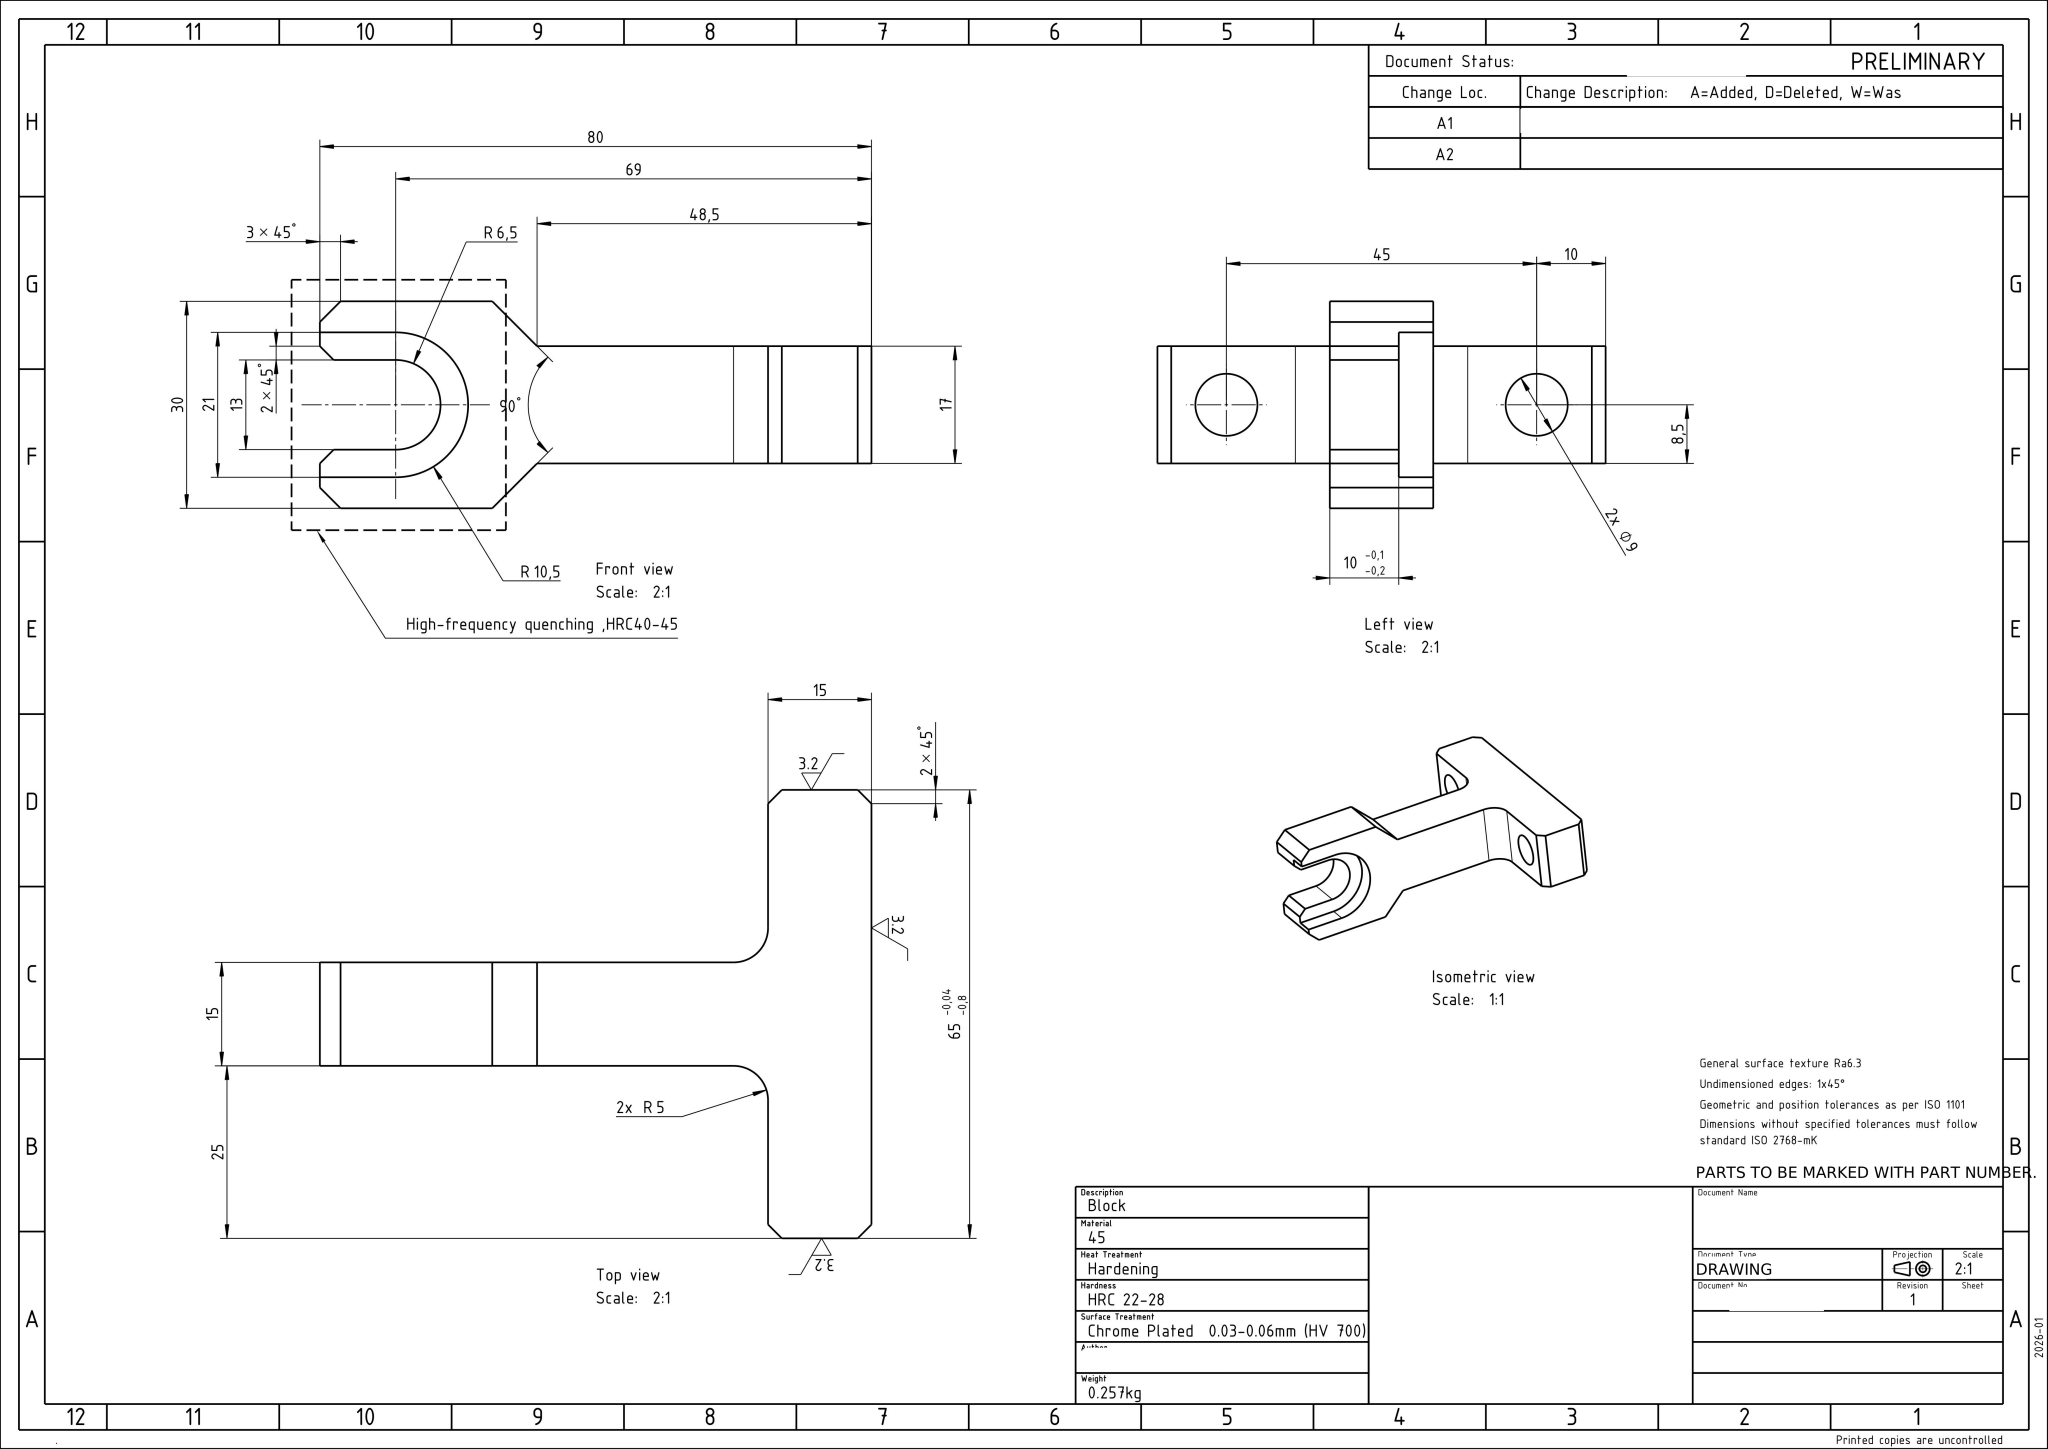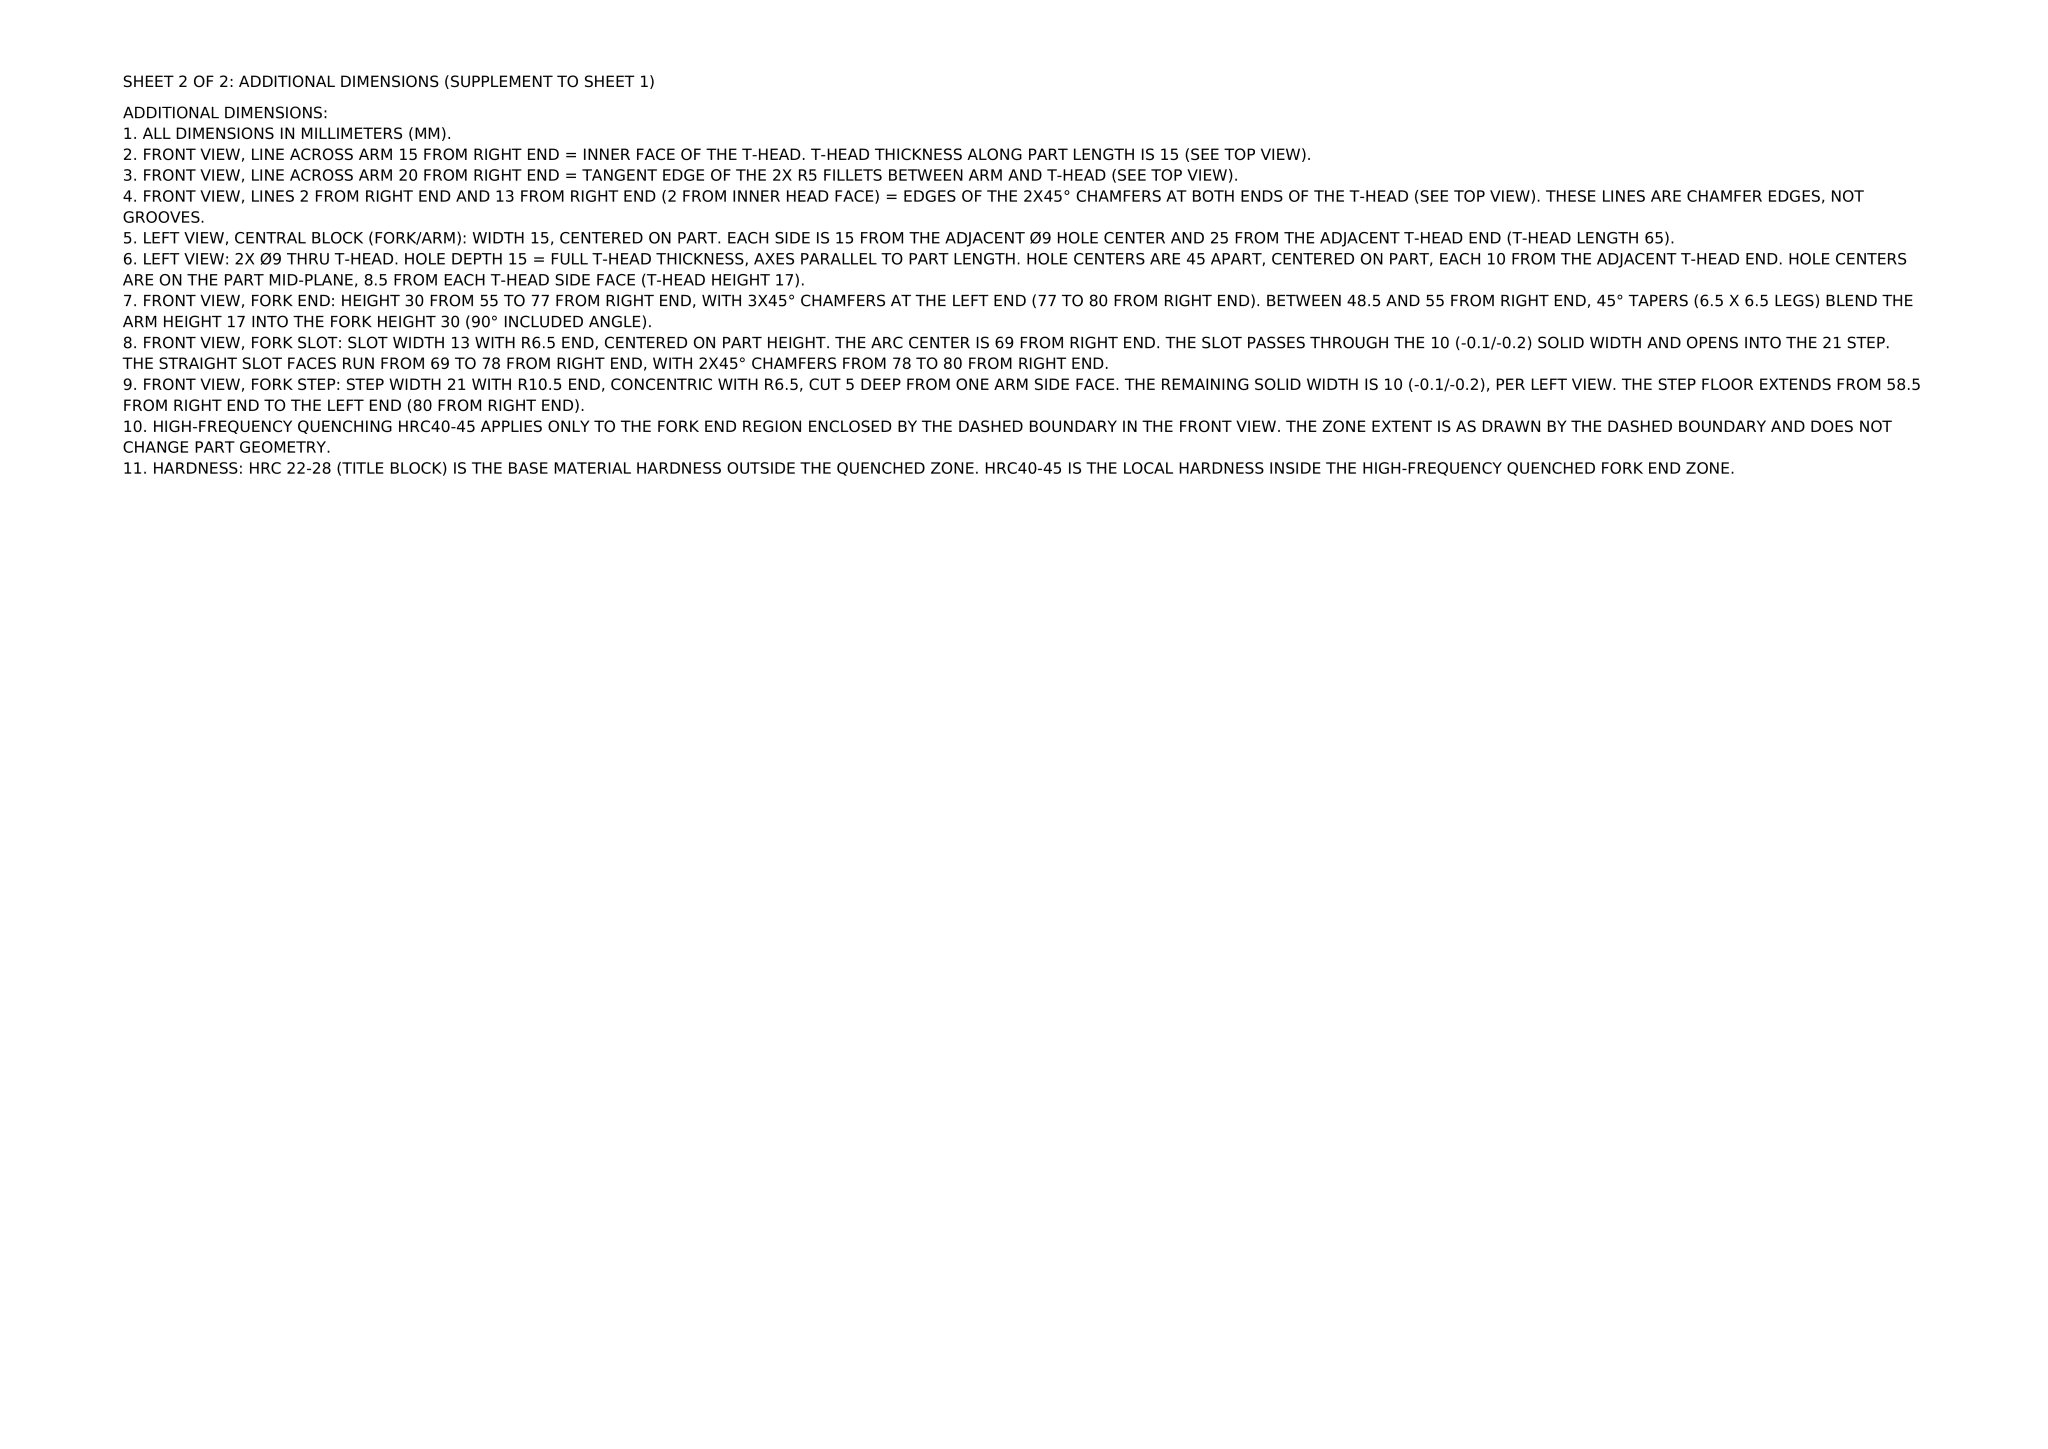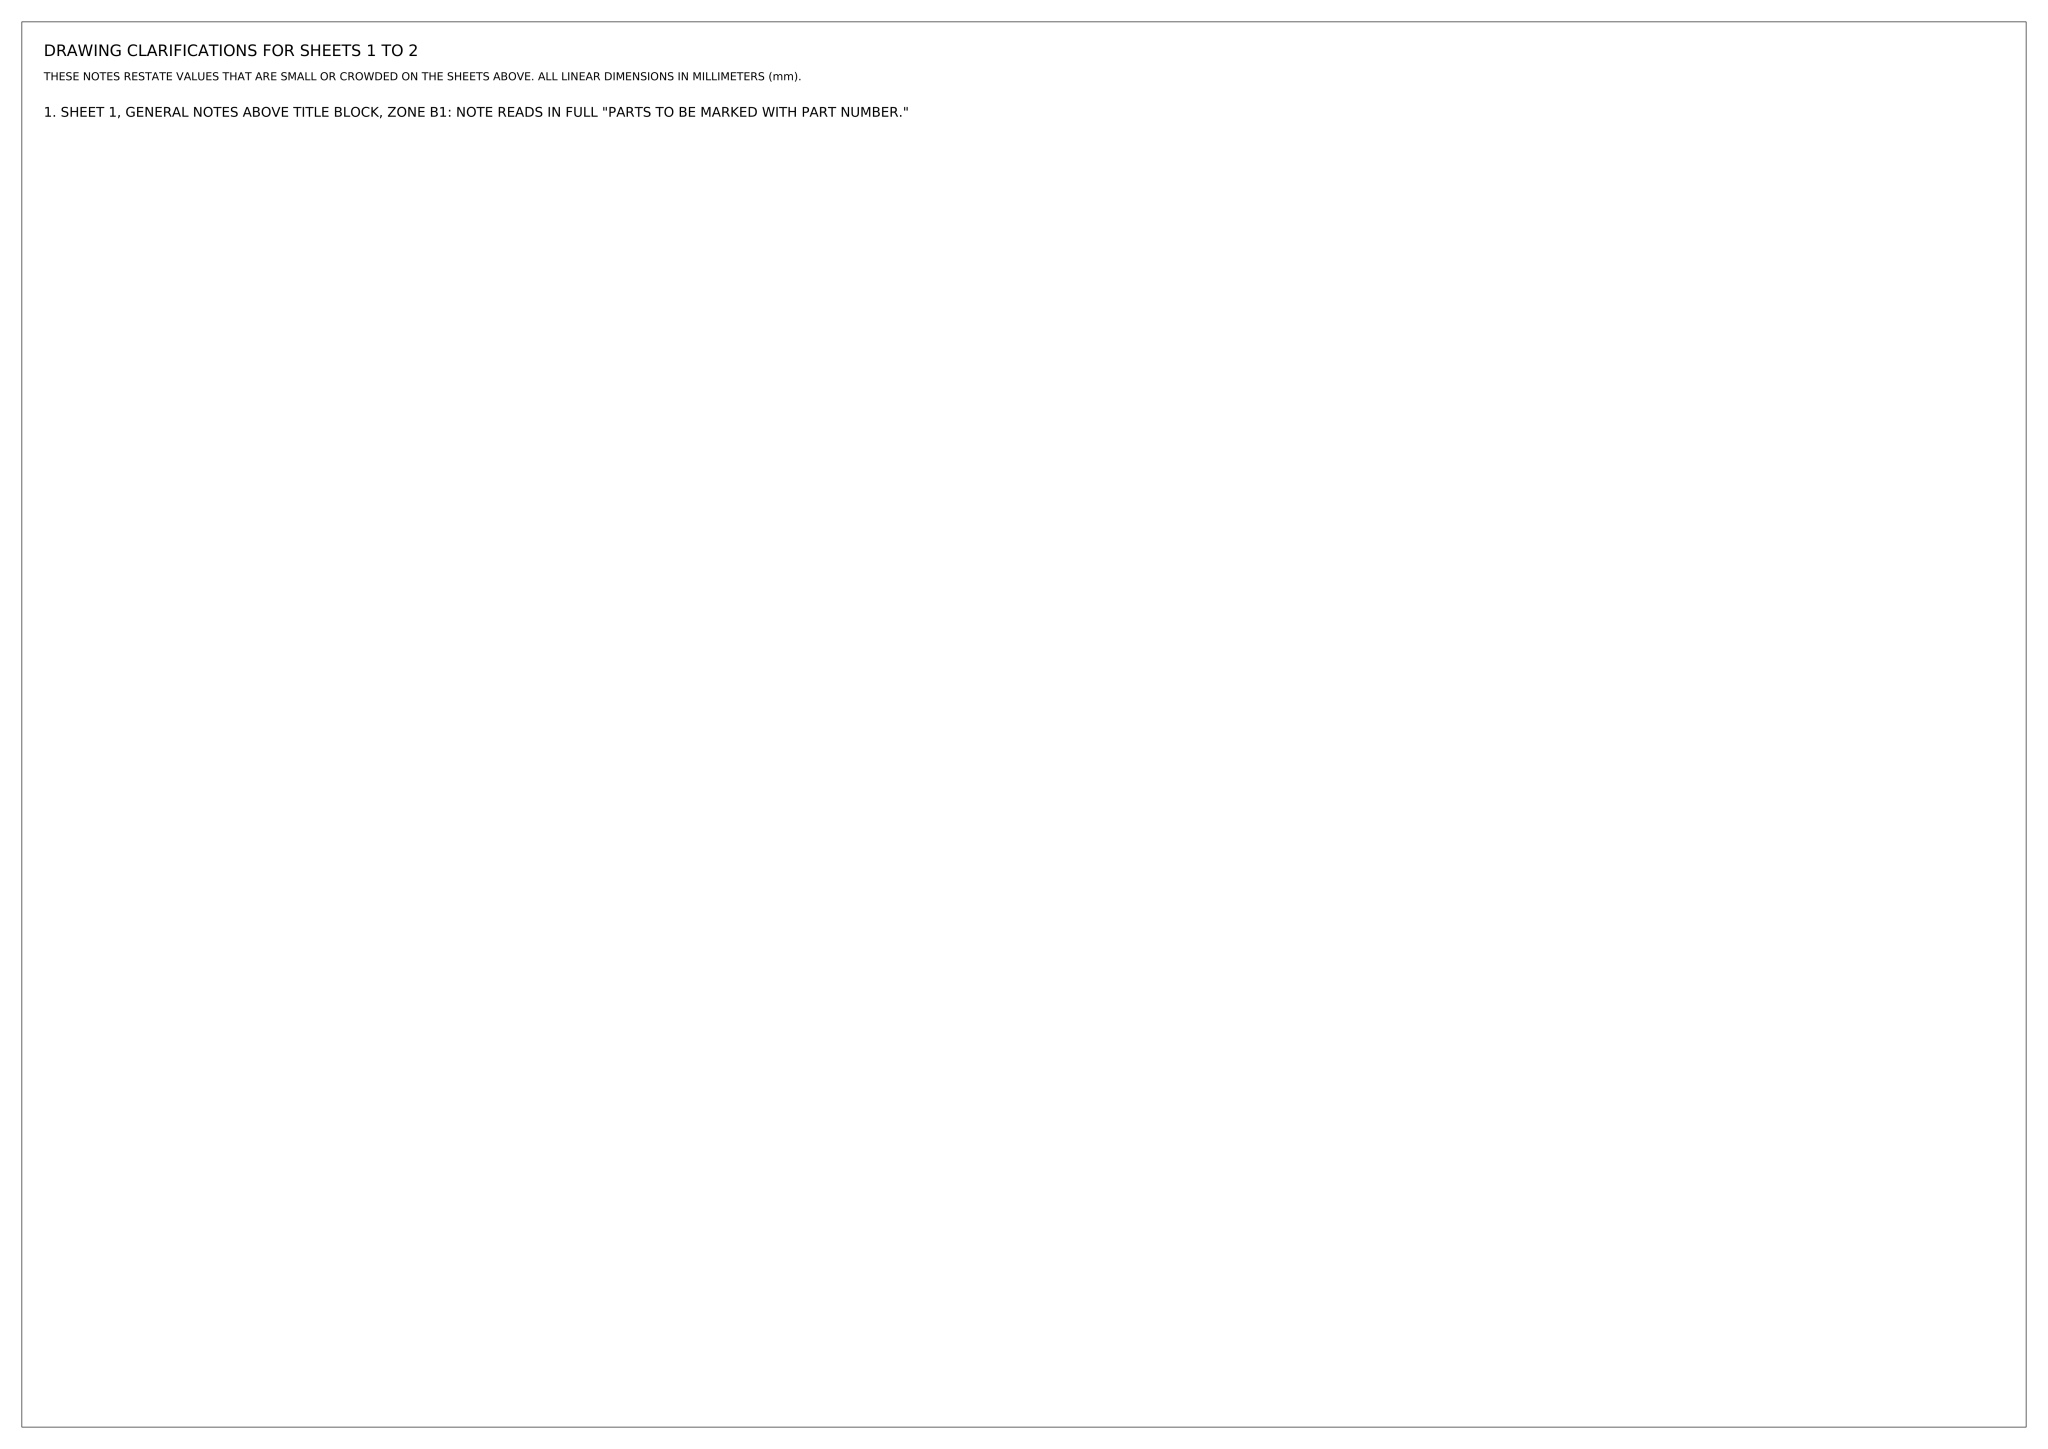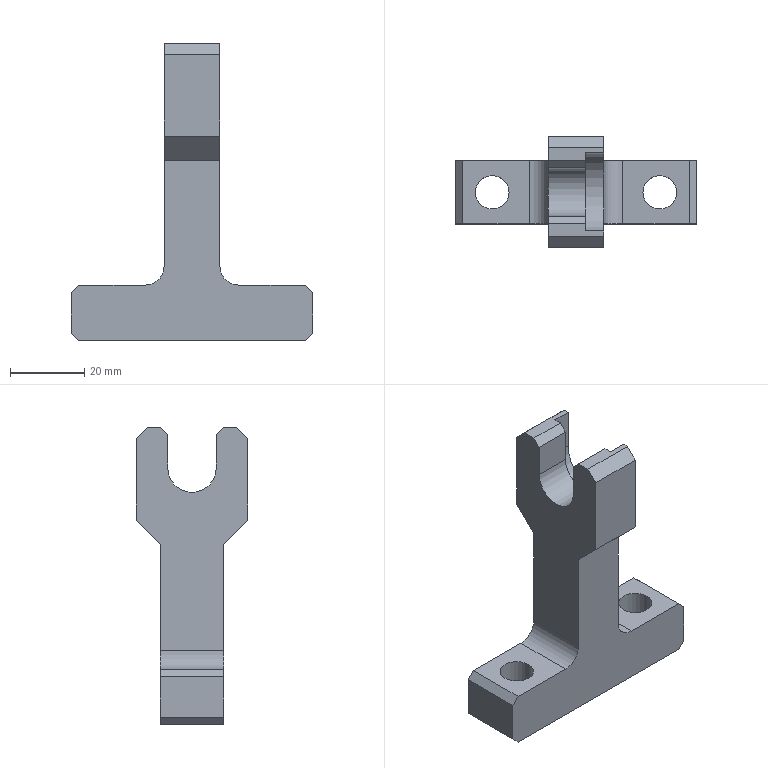Part | NX | mm | 1 solid | 34 faces | box 65 x 30 x 80 mm | volume 32507 mm3 | plane 28 | cylinder 6 | commonest cylinder face diameters 10 x2 9 x2 13 x1 21 x1